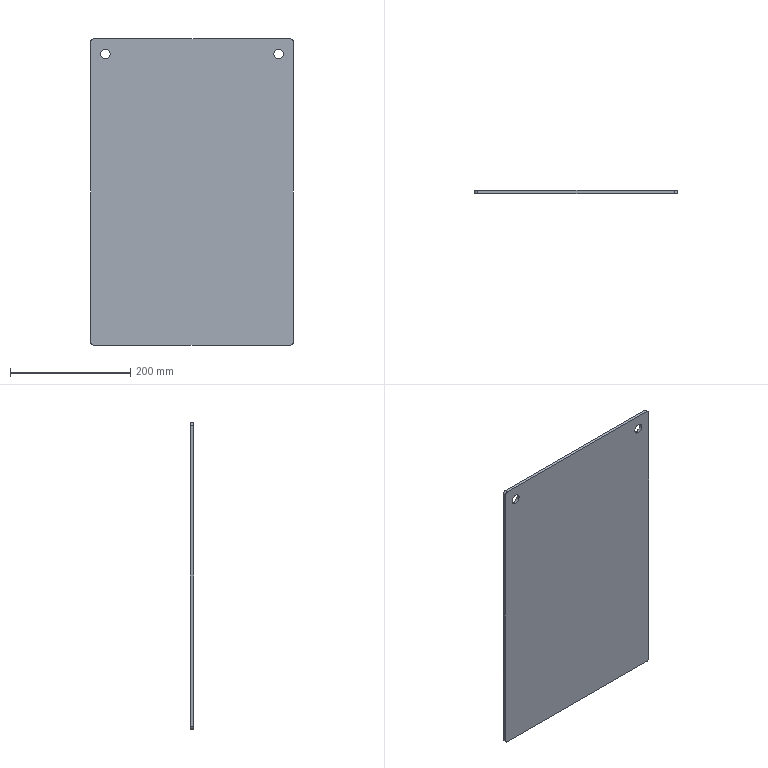Component | SolidWorks | 008FrameTopCoverPlate-1 | 1 solid | 14 faces | box 338 x 5 x 510 mm | volume 859661 mm3 | plane 6 | cone 4 | cylinder 4 | commonest cylinder face diameters 10 x4 | material Plain Carbon Steel
build123d program:
from build123d import *

# Parameters (mm, degrees)
SKETCH1_W                        = 510
SKETCH1_H                        = 338
BOSS_EXTRUDE1_DEPTH              = 5
FILLET1_R                        = 5
F_1_2_RC_TAPPED_HOLE1_AT_2_COUNT = 2
F_1_2_RC_TAPPED_HOLE1_AT_2_PITCH = 289


with BuildPart() as part:
    # Sketch1 → Boss-Extrude1 (new body)
    with BuildSketch(Plane.XY):
        Rectangle(SKETCH1_W, SKETCH1_H)
    extrude(amount=BOSS_EXTRUDE1_DEPTH)

    # Fillet1
    fillet1_edges = [part.edges().sort_by_distance(p)[0] for p in [
        (255, -169, 2.5),
        (-255, -169, 2.5),
        (-255, 169, 2.5),
        (255, 169, 2.5),
    ]]
    fillet(fillet1_edges, radius=FILLET1_R)

    # Sketch2 → 1_2 Rc Tapped Hole1 (revolve, cut)
    with BuildSketch(Plane(origin=(-230, -144.5, 0), x_dir=(0, 1, 0), z_dir=(1, 0, 0))):
        Polygon((0, 0), (0, 29.328), (8.75, 24.07), (8.75, 15), (7.847, 15), (8.316, 0), align=None)
    f_1_2_rc_tapped_hole1 = revolve(axis=Axis((-230, -144.5, -6.35), (0, 0, 1)), mode=Mode.SUBTRACT)

    # 1_2 Rc Tapped Hole1 at 2: 1_2 Rc Tapped Hole1 ×2
    with Locations(*[(0, i * F_1_2_RC_TAPPED_HOLE1_AT_2_PITCH, 0) for i in range(1, F_1_2_RC_TAPPED_HOLE1_AT_2_COUNT)]):
        add(f_1_2_rc_tapped_hole1, mode=Mode.SUBTRACT)


solid = part.part

# Placed as in the assembly
solid = solid.moved(Location((130, 1377, -260), (90, 0, -90)))
STEP:
#1=COLOUR_RGB('',0.7922,0.8196,0.9333);
#2=FILL_AREA_STYLE_COLOUR('',#1);
#3=FILL_AREA_STYLE('',(#2));
#4=SURFACE_STYLE_FILL_AREA(#3);
#5=SURFACE_SIDE_STYLE('',(#4));
#6=SURFACE_STYLE_USAGE(.BOTH.,#5);
#7=PRESENTATION_STYLE_ASSIGNMENT((#6));
#8=CARTESIAN_POINT('',(-0.5709,54.016,-1.502));
#9=VERTEX_POINT('',#8);
#10=CARTESIAN_POINT('',(-0.5709,54.016,-0.8599));
#11=VERTEX_POINT('',#10);
#12=CARTESIAN_POINT('',(-0.5709,54.016,-1.181));
#13=DIRECTION('',(0.,1.,0.));
#14=DIRECTION('',(-0.,0.,1.));
#15=AXIS2_PLACEMENT_3D('',#12,#13,#14);
#16=CIRCLE('',#15,0.3212);
#17=EDGE_CURVE('',#9,#11,#16,.T.);
#18=ORIENTED_EDGE('',*,*,#17,.F.);
#19=CARTESIAN_POINT('',(-0.5709,54.213,-1.508));
#20=VERTEX_POINT('',#19);
#21=CARTESIAN_POINT('',(-0.5709,54.213,-1.508));
#22=DIRECTION('',(0.,0.9995,-0.0312));
#23=VECTOR('',#22,39.37);
#24=LINE('',#21,#23);
#25=EDGE_CURVE('',#9,#20,#24,.T.);
#26=ORIENTED_EDGE('',*,*,#25,.T.);
#27=CARTESIAN_POINT('',(-0.5709,54.213,-0.8537));
#28=VERTEX_POINT('',#27);
#29=CARTESIAN_POINT('',(-0.5709,54.213,-1.181));
#30=DIRECTION('',(0.,1.,0.));
#31=DIRECTION('',(-0.,0.,1.));
#32=AXIS2_PLACEMENT_3D('',#29,#30,#31);
#33=CIRCLE('',#32,0.3274);
#34=EDGE_CURVE('',#20,#28,#33,.T.);
#35=ORIENTED_EDGE('',*,*,#34,.T.);
#36=CARTESIAN_POINT('',(-0.5709,54.213,-0.8537));
#37=DIRECTION('',(-0.,0.9995,0.0312));
#38=VECTOR('',#37,39.37);
#39=LINE('',#36,#38);
#40=EDGE_CURVE('',#11,#28,#39,.T.);
#41=ORIENTED_EDGE('',*,*,#40,.F.);
#42=EDGE_LOOP('',(#18,#26,#35,#41));
#43=FACE_OUTER_BOUND('',#42,.T.);
#44=CARTESIAN_POINT('',(-0.5709,54.213,-1.181));
#45=DIRECTION('',(0.,1.,0.));
#46=DIRECTION('',(-0.,0.,1.));
#47=AXIS2_PLACEMENT_3D('',#44,#45,#46);
#48=CONICAL_SURFACE('',#47,0.3274,0.03121);
#49=ADVANCED_FACE('',(#43),#48,.F.);
#50=CARTESIAN_POINT('',(10.807,54.016,-1.502));
#51=VERTEX_POINT('',#50);
#52=CARTESIAN_POINT('',(10.807,54.016,-0.8599));
#53=VERTEX_POINT('',#52);
#54=CARTESIAN_POINT('',(10.807,54.016,-1.181));
#55=DIRECTION('',(0.,1.,0.));
#56=DIRECTION('',(0.,0.,1.));
#57=AXIS2_PLACEMENT_3D('',#54,#55,#56);
#58=CIRCLE('',#57,0.3212);
#59=EDGE_CURVE('',#51,#53,#58,.T.);
#60=ORIENTED_EDGE('',*,*,#59,.F.);
#61=CARTESIAN_POINT('',(10.807,54.213,-1.508));
#62=VERTEX_POINT('',#61);
#63=CARTESIAN_POINT('',(10.807,54.213,-1.508));
#64=DIRECTION('',(0.,0.9995,-0.0312));
#65=VECTOR('',#64,39.37);
#66=LINE('',#63,#65);
#67=EDGE_CURVE('',#51,#62,#66,.T.);
#68=ORIENTED_EDGE('',*,*,#67,.T.);
#69=CARTESIAN_POINT('',(10.807,54.213,-0.8537));
#70=VERTEX_POINT('',#69);
#71=CARTESIAN_POINT('',(10.807,54.213,-1.181));
#72=DIRECTION('',(0.,1.,0.));
#73=DIRECTION('',(0.,0.,1.));
#74=AXIS2_PLACEMENT_3D('',#71,#72,#73);
#75=CIRCLE('',#74,0.3274);
#76=EDGE_CURVE('',#62,#70,#75,.T.);
#77=ORIENTED_EDGE('',*,*,#76,.T.);
#78=CARTESIAN_POINT('',(10.807,54.213,-0.8537));
#79=DIRECTION('',(-0.,0.9995,0.0312));
#80=VECTOR('',#79,39.37);
#81=LINE('',#78,#80);
#82=EDGE_CURVE('',#53,#70,#81,.T.);
#83=ORIENTED_EDGE('',*,*,#82,.F.);
#84=EDGE_LOOP('',(#60,#68,#77,#83));
#85=FACE_OUTER_BOUND('',#84,.T.);
#86=CARTESIAN_POINT('',(10.807,54.213,-1.181));
#87=DIRECTION('',(0.,1.,0.));
#88=DIRECTION('',(0.,0.,1.));
#89=AXIS2_PLACEMENT_3D('',#86,#87,#88);
#90=CONICAL_SURFACE('',#89,0.3274,0.03121);
#91=ADVANCED_FACE('',(#85),#90,.F.);
#92=CARTESIAN_POINT('',(-1.339,54.016,-20.276));
#93=VERTEX_POINT('',#92);
#94=CARTESIAN_POINT('',(11.575,54.016,-20.276));
#95=VERTEX_POINT('',#94);
#96=CARTESIAN_POINT('',(-1.535,54.016,-20.276));
#97=DIRECTION('',(1.,0.,0.));
#98=VECTOR('',#97,39.37);
#99=LINE('',#96,#98);
#100=EDGE_CURVE('',#93,#95,#99,.T.);
#101=ORIENTED_EDGE('',*,*,#100,.F.);
#102=CARTESIAN_POINT('',(-1.339,54.213,-20.276));
#103=VERTEX_POINT('',#102);
#104=CARTESIAN_POINT('',(-1.339,54.016,-20.276));
#105=DIRECTION('',(0.,1.,0.));
#106=VECTOR('',#105,39.37);
#107=LINE('',#104,#106);
#108=EDGE_CURVE('',#93,#103,#107,.T.);
#109=ORIENTED_EDGE('',*,*,#108,.T.);
#110=CARTESIAN_POINT('',(11.575,54.213,-20.276));
#111=VERTEX_POINT('',#110);
#112=CARTESIAN_POINT('',(-1.535,54.213,-20.276));
#113=DIRECTION('',(1.,0.,0.));
#114=VECTOR('',#113,39.37);
#115=LINE('',#112,#114);
#116=EDGE_CURVE('',#103,#111,#115,.T.);
#117=ORIENTED_EDGE('',*,*,#116,.T.);
#118=CARTESIAN_POINT('',(11.575,54.016,-20.276));
#119=DIRECTION('',(0.,-1.,0.));
#120=VECTOR('',#119,39.37);
#121=LINE('',#118,#120);
#122=EDGE_CURVE('',#111,#95,#121,.T.);
#123=ORIENTED_EDGE('',*,*,#122,.T.);
#124=EDGE_LOOP('',(#101,#109,#117,#123));
#125=FACE_OUTER_BOUND('',#124,.T.);
#126=CARTESIAN_POINT('',(-1.535,54.016,-20.276));
#127=DIRECTION('',(-0.,0.,1.));
#128=DIRECTION('',(0.,-1.,0.));
#129=AXIS2_PLACEMENT_3D('',#126,#127,#128);
#130=PLANE('',#129);
#131=ADVANCED_FACE('',(#125),#130,.F.);
#132=CARTESIAN_POINT('',(11.772,54.213,-20.079));
#133=VERTEX_POINT('',#132);
#134=CARTESIAN_POINT('',(11.772,54.213,-0.3937));
#135=VERTEX_POINT('',#134);
#136=CARTESIAN_POINT('',(11.772,54.213,-0.1969));
#137=DIRECTION('',(-0.,0.,1.));
#138=VECTOR('',#137,39.37);
#139=LINE('',#136,#138);
#140=EDGE_CURVE('',#133,#135,#139,.T.);
#141=ORIENTED_EDGE('',*,*,#140,.T.);
#142=CARTESIAN_POINT('',(11.772,54.016,-0.3937));
#143=VERTEX_POINT('',#142);
#144=CARTESIAN_POINT('',(11.772,54.016,-0.3937));
#145=DIRECTION('',(0.,-1.,0.));
#146=VECTOR('',#145,39.37);
#147=LINE('',#144,#146);
#148=EDGE_CURVE('',#135,#143,#147,.T.);
#149=ORIENTED_EDGE('',*,*,#148,.T.);
#150=CARTESIAN_POINT('',(11.772,54.016,-20.079));
#151=VERTEX_POINT('',#150);
#152=CARTESIAN_POINT('',(11.772,54.016,-0.1969));
#153=DIRECTION('',(-0.,0.,1.));
#154=VECTOR('',#153,39.37);
#155=LINE('',#152,#154);
#156=EDGE_CURVE('',#151,#143,#155,.T.);
#157=ORIENTED_EDGE('',*,*,#156,.F.);
#158=CARTESIAN_POINT('',(11.772,54.016,-20.079));
#159=DIRECTION('',(0.,1.,0.));
#160=VECTOR('',#159,39.37);
#161=LINE('',#158,#160);
#162=EDGE_CURVE('',#151,#133,#161,.T.);
#163=ORIENTED_EDGE('',*,*,#162,.T.);
#164=EDGE_LOOP('',(#141,#149,#157,#163));
#165=FACE_OUTER_BOUND('',#164,.T.);
#166=CARTESIAN_POINT('',(11.772,54.016,-0.1969));
#167=DIRECTION('',(-1.,0.,-0.));
#168=DIRECTION('',(0.,1.,0.));
#169=AXIS2_PLACEMENT_3D('',#166,#167,#168);
#170=PLANE('',#169);
#171=ADVANCED_FACE('',(#165),#170,.F.);
#172=CARTESIAN_POINT('',(11.575,54.213,-0.1969));
#173=VERTEX_POINT('',#172);
#174=CARTESIAN_POINT('',(-1.339,54.213,-0.1969));
#175=VERTEX_POINT('',#174);
#176=CARTESIAN_POINT('',(-1.535,54.213,-0.1969));
#177=DIRECTION('',(-1.,0.,-0.));
#178=VECTOR('',#177,39.37);
#179=LINE('',#176,#178);
#180=EDGE_CURVE('',#173,#175,#179,.T.);
#181=ORIENTED_EDGE('',*,*,#180,.T.);
#182=CARTESIAN_POINT('',(-1.339,54.016,-0.1969));
#183=VERTEX_POINT('',#182);
#184=CARTESIAN_POINT('',(-1.339,54.016,-0.1969));
#185=DIRECTION('',(0.,-1.,0.));
#186=VECTOR('',#185,39.37);
#187=LINE('',#184,#186);
#188=EDGE_CURVE('',#175,#183,#187,.T.);
#189=ORIENTED_EDGE('',*,*,#188,.T.);
#190=CARTESIAN_POINT('',(11.575,54.016,-0.1969));
#191=VERTEX_POINT('',#190);
#192=CARTESIAN_POINT('',(-1.535,54.016,-0.1969));
#193=DIRECTION('',(-1.,0.,-0.));
#194=VECTOR('',#193,39.37);
#195=LINE('',#192,#194);
#196=EDGE_CURVE('',#191,#183,#195,.T.);
#197=ORIENTED_EDGE('',*,*,#196,.F.);
#198=CARTESIAN_POINT('',(11.575,54.016,-0.1969));
#199=DIRECTION('',(0.,1.,0.));
#200=VECTOR('',#199,39.37);
#201=LINE('',#198,#200);
#202=EDGE_CURVE('',#191,#173,#201,.T.);
#203=ORIENTED_EDGE('',*,*,#202,.T.);
#204=EDGE_LOOP('',(#181,#189,#197,#203));
#205=FACE_OUTER_BOUND('',#204,.T.);
#206=CARTESIAN_POINT('',(-1.535,54.016,-0.1969));
#207=DIRECTION('',(0.,0.,-1.));
#208=DIRECTION('',(0.,1.,0.));
#209=AXIS2_PLACEMENT_3D('',#206,#207,#208);
#210=PLANE('',#209);
#211=ADVANCED_FACE('',(#205),#210,.F.);
#212=CARTESIAN_POINT('',(-1.535,54.213,-0.3937));
#213=VERTEX_POINT('',#212);
#214=CARTESIAN_POINT('',(-1.535,54.213,-20.079));
#215=VERTEX_POINT('',#214);
#216=CARTESIAN_POINT('',(-1.535,54.213,-0.1969));
#217=DIRECTION('',(0.,0.,-1.));
#218=VECTOR('',#217,39.37);
#219=LINE('',#216,#218);
#220=EDGE_CURVE('',#213,#215,#219,.T.);
#221=ORIENTED_EDGE('',*,*,#220,.T.);
#222=CARTESIAN_POINT('',(-1.535,54.016,-20.079));
#223=VERTEX_POINT('',#222);
#224=CARTESIAN_POINT('',(-1.535,54.016,-20.079));
#225=DIRECTION('',(0.,-1.,0.));
#226=VECTOR('',#225,39.37);
#227=LINE('',#224,#226);
#228=EDGE_CURVE('',#215,#223,#227,.T.);
#229=ORIENTED_EDGE('',*,*,#228,.T.);
#230=CARTESIAN_POINT('',(-1.535,54.016,-0.3937));
#231=VERTEX_POINT('',#230);
#232=CARTESIAN_POINT('',(-1.535,54.016,-0.1969));
#233=DIRECTION('',(0.,0.,-1.));
#234=VECTOR('',#233,39.37);
#235=LINE('',#232,#234);
#236=EDGE_CURVE('',#231,#223,#235,.T.);
#237=ORIENTED_EDGE('',*,*,#236,.F.);
#238=CARTESIAN_POINT('',(-1.535,54.016,-0.3937));
#239=DIRECTION('',(0.,1.,0.));
#240=VECTOR('',#239,39.37);
#241=LINE('',#238,#240);
#242=EDGE_CURVE('',#231,#213,#241,.T.);
#243=ORIENTED_EDGE('',*,*,#242,.T.);
#244=EDGE_LOOP('',(#221,#229,#237,#243));
#245=FACE_OUTER_BOUND('',#244,.T.);
#246=CARTESIAN_POINT('',(-1.535,54.016,-0.1969));
#247=DIRECTION('',(1.,0.,0.));
#248=DIRECTION('',(0.,-1.,0.));
#249=AXIS2_PLACEMENT_3D('',#246,#247,#248);
#250=PLANE('',#249);
#251=ADVANCED_FACE('',(#245),#250,.F.);
#252=CARTESIAN_POINT('',(-0.5709,54.016,-1.181));
#253=DIRECTION('',(0.,1.,0.));
#254=DIRECTION('',(-0.,0.,1.));
#255=AXIS2_PLACEMENT_3D('',#252,#253,#254);
#256=CIRCLE('',#255,0.3212);
#257=EDGE_CURVE('',#11,#9,#256,.T.);
#258=ORIENTED_EDGE('',*,*,#257,.T.);
#259=ORIENTED_EDGE('',*,*,#17,.T.);
#260=EDGE_LOOP('',(#258,#259));
#261=FACE_BOUND('',#260,.T.);
#262=CARTESIAN_POINT('',(10.807,54.016,-1.181));
#263=DIRECTION('',(0.,1.,0.));
#264=DIRECTION('',(0.,0.,1.));
#265=AXIS2_PLACEMENT_3D('',#262,#263,#264);
#266=CIRCLE('',#265,0.3212);
#267=EDGE_CURVE('',#53,#51,#266,.T.);
#268=ORIENTED_EDGE('',*,*,#267,.T.);
#269=ORIENTED_EDGE('',*,*,#59,.T.);
#270=EDGE_LOOP('',(#268,#269));
#271=FACE_BOUND('',#270,.T.);
#272=ORIENTED_EDGE('',*,*,#236,.T.);
#273=CARTESIAN_POINT('',(-1.339,54.016,-20.079));
#274=DIRECTION('',(0.,-1.,0.));
#275=DIRECTION('',(0.,0.,1.));
#276=AXIS2_PLACEMENT_3D('',#273,#274,#275);
#277=CIRCLE('',#276,0.1969);
#278=EDGE_CURVE('',#223,#93,#277,.T.);
#279=ORIENTED_EDGE('',*,*,#278,.T.);
#280=ORIENTED_EDGE('',*,*,#100,.T.);
#281=CARTESIAN_POINT('',(11.575,54.016,-20.079));
#282=DIRECTION('',(0.,-1.,0.));
#283=DIRECTION('',(0.,0.,1.));
#284=AXIS2_PLACEMENT_3D('',#281,#282,#283);
#285=CIRCLE('',#284,0.1969);
#286=EDGE_CURVE('',#95,#151,#285,.T.);
#287=ORIENTED_EDGE('',*,*,#286,.T.);
#288=ORIENTED_EDGE('',*,*,#156,.T.);
#289=CARTESIAN_POINT('',(11.575,54.016,-0.3937));
#290=DIRECTION('',(0.,-1.,0.));
#291=DIRECTION('',(0.,0.,1.));
#292=AXIS2_PLACEMENT_3D('',#289,#290,#291);
#293=CIRCLE('',#292,0.1969);
#294=EDGE_CURVE('',#143,#191,#293,.T.);
#295=ORIENTED_EDGE('',*,*,#294,.T.);
#296=ORIENTED_EDGE('',*,*,#196,.T.);
#297=CARTESIAN_POINT('',(-1.339,54.016,-0.3937));
#298=DIRECTION('',(0.,-1.,0.));
#299=DIRECTION('',(0.,0.,1.));
#300=AXIS2_PLACEMENT_3D('',#297,#298,#299);
#301=CIRCLE('',#300,0.1969);
#302=EDGE_CURVE('',#183,#231,#301,.T.);
#303=ORIENTED_EDGE('',*,*,#302,.T.);
#304=EDGE_LOOP('',(#272,#279,#280,#287,#288,#295,#296,#303));
#305=FACE_OUTER_BOUND('',#304,.T.);
#306=CARTESIAN_POINT('',(11.772,54.016,-20.276));
#307=DIRECTION('',(0.,1.,0.));
#308=DIRECTION('',(-0.,0.,1.));
#309=AXIS2_PLACEMENT_3D('',#306,#307,#308);
#310=PLANE('',#309);
#311=ADVANCED_FACE('',(#261,#271,#305),#310,.F.);
#312=CARTESIAN_POINT('',(-0.5709,54.213,-1.181));
#313=DIRECTION('',(0.,1.,0.));
#314=DIRECTION('',(-0.,0.,1.));
#315=AXIS2_PLACEMENT_3D('',#312,#313,#314);
#316=CIRCLE('',#315,0.3274);
#317=EDGE_CURVE('',#28,#20,#316,.T.);
#318=ORIENTED_EDGE('',*,*,#317,.F.);
#319=ORIENTED_EDGE('',*,*,#34,.F.);
#320=EDGE_LOOP('',(#318,#319));
#321=FACE_BOUND('',#320,.T.);
#322=CARTESIAN_POINT('',(10.807,54.213,-1.181));
#323=DIRECTION('',(0.,1.,0.));
#324=DIRECTION('',(0.,0.,1.));
#325=AXIS2_PLACEMENT_3D('',#322,#323,#324);
#326=CIRCLE('',#325,0.3274);
#327=EDGE_CURVE('',#70,#62,#326,.T.);
#328=ORIENTED_EDGE('',*,*,#327,.F.);
#329=ORIENTED_EDGE('',*,*,#76,.F.);
#330=EDGE_LOOP('',(#328,#329));
#331=FACE_BOUND('',#330,.T.);
#332=ORIENTED_EDGE('',*,*,#116,.F.);
#333=CARTESIAN_POINT('',(-1.339,54.213,-20.079));
#334=DIRECTION('',(0.,1.,0.));
#335=DIRECTION('',(0.,0.,1.));
#336=AXIS2_PLACEMENT_3D('',#333,#334,#335);
#337=CIRCLE('',#336,0.1969);
#338=EDGE_CURVE('',#103,#215,#337,.T.);
#339=ORIENTED_EDGE('',*,*,#338,.T.);
#340=ORIENTED_EDGE('',*,*,#220,.F.);
#341=CARTESIAN_POINT('',(-1.339,54.213,-0.3937));
#342=DIRECTION('',(0.,1.,0.));
#343=DIRECTION('',(0.,0.,1.));
#344=AXIS2_PLACEMENT_3D('',#341,#342,#343);
#345=CIRCLE('',#344,0.1969);
#346=EDGE_CURVE('',#213,#175,#345,.T.);
#347=ORIENTED_EDGE('',*,*,#346,.T.);
#348=ORIENTED_EDGE('',*,*,#180,.F.);
#349=CARTESIAN_POINT('',(11.575,54.213,-0.3937));
#350=DIRECTION('',(0.,1.,0.));
#351=DIRECTION('',(0.,0.,1.));
#352=AXIS2_PLACEMENT_3D('',#349,#350,#351);
#353=CIRCLE('',#352,0.1969);
#354=EDGE_CURVE('',#173,#135,#353,.T.);
#355=ORIENTED_EDGE('',*,*,#354,.T.);
#356=ORIENTED_EDGE('',*,*,#140,.F.);
#357=CARTESIAN_POINT('',(11.575,54.213,-20.079));
#358=DIRECTION('',(0.,1.,0.));
#359=DIRECTION('',(0.,0.,1.));
#360=AXIS2_PLACEMENT_3D('',#357,#358,#359);
#361=CIRCLE('',#360,0.1969);
#362=EDGE_CURVE('',#133,#111,#361,.T.);
#363=ORIENTED_EDGE('',*,*,#362,.T.);
#364=EDGE_LOOP('',(#332,#339,#340,#347,#348,#355,#356,#363));
#365=FACE_OUTER_BOUND('',#364,.T.);
#366=CARTESIAN_POINT('',(11.772,54.213,-20.276));
#367=DIRECTION('',(0.,1.,0.));
#368=DIRECTION('',(-0.,0.,1.));
#369=AXIS2_PLACEMENT_3D('',#366,#367,#368);
#370=PLANE('',#369);
#371=ADVANCED_FACE('',(#321,#331,#365),#370,.T.);
#372=ORIENTED_EDGE('',*,*,#278,.F.);
#373=ORIENTED_EDGE('',*,*,#228,.F.);
#374=ORIENTED_EDGE('',*,*,#338,.F.);
#375=ORIENTED_EDGE('',*,*,#108,.F.);
#376=EDGE_LOOP('',(#372,#373,#374,#375));
#377=FACE_OUTER_BOUND('',#376,.T.);
#378=CARTESIAN_POINT('',(-1.339,54.016,-20.079));
#379=DIRECTION('',(0.,1.,0.));
#380=DIRECTION('',(0.,0.,1.));
#381=AXIS2_PLACEMENT_3D('',#378,#379,#380);
#382=CYLINDRICAL_SURFACE('',#381,0.1969);
#383=ADVANCED_FACE('',(#377),#382,.T.);
#384=ORIENTED_EDGE('',*,*,#302,.F.);
#385=ORIENTED_EDGE('',*,*,#188,.F.);
#386=ORIENTED_EDGE('',*,*,#346,.F.);
#387=ORIENTED_EDGE('',*,*,#242,.F.);
#388=EDGE_LOOP('',(#384,#385,#386,#387));
#389=FACE_OUTER_BOUND('',#388,.T.);
#390=CARTESIAN_POINT('',(-1.339,54.016,-0.3937));
#391=DIRECTION('',(0.,1.,0.));
#392=DIRECTION('',(0.,0.,1.));
#393=AXIS2_PLACEMENT_3D('',#390,#391,#392);
#394=CYLINDRICAL_SURFACE('',#393,0.1969);
#395=ADVANCED_FACE('',(#389),#394,.T.);
#396=ORIENTED_EDGE('',*,*,#294,.F.);
#397=ORIENTED_EDGE('',*,*,#148,.F.);
#398=ORIENTED_EDGE('',*,*,#354,.F.);
#399=ORIENTED_EDGE('',*,*,#202,.F.);
#400=EDGE_LOOP('',(#396,#397,#398,#399));
#401=FACE_OUTER_BOUND('',#400,.T.);
#402=CARTESIAN_POINT('',(11.575,54.016,-0.3937));
#403=DIRECTION('',(0.,1.,0.));
#404=DIRECTION('',(0.,0.,1.));
#405=AXIS2_PLACEMENT_3D('',#402,#403,#404);
#406=CYLINDRICAL_SURFACE('',#405,0.1969);
#407=ADVANCED_FACE('',(#401),#406,.T.);
#408=ORIENTED_EDGE('',*,*,#286,.F.);
#409=ORIENTED_EDGE('',*,*,#122,.F.);
#410=ORIENTED_EDGE('',*,*,#362,.F.);
#411=ORIENTED_EDGE('',*,*,#162,.F.);
#412=EDGE_LOOP('',(#408,#409,#410,#411));
#413=FACE_OUTER_BOUND('',#412,.T.);
#414=CARTESIAN_POINT('',(11.575,54.016,-20.079));
#415=DIRECTION('',(0.,1.,0.));
#416=DIRECTION('',(0.,0.,1.));
#417=AXIS2_PLACEMENT_3D('',#414,#415,#416);
#418=CYLINDRICAL_SURFACE('',#417,0.1969);
#419=ADVANCED_FACE('',(#413),#418,.T.);
#420=ORIENTED_EDGE('',*,*,#67,.F.);
#421=ORIENTED_EDGE('',*,*,#267,.F.);
#422=ORIENTED_EDGE('',*,*,#82,.T.);
#423=ORIENTED_EDGE('',*,*,#327,.T.);
#424=EDGE_LOOP('',(#420,#421,#422,#423));
#425=FACE_OUTER_BOUND('',#424,.T.);
#426=CARTESIAN_POINT('',(10.807,54.213,-1.181));
#427=DIRECTION('',(0.,1.,0.));
#428=DIRECTION('',(0.,0.,1.));
#429=AXIS2_PLACEMENT_3D('',#426,#427,#428);
#430=CONICAL_SURFACE('',#429,0.3274,0.03121);
#431=ADVANCED_FACE('',(#425),#430,.F.);
#432=ORIENTED_EDGE('',*,*,#25,.F.);
#433=ORIENTED_EDGE('',*,*,#257,.F.);
#434=ORIENTED_EDGE('',*,*,#40,.T.);
#435=ORIENTED_EDGE('',*,*,#317,.T.);
#436=EDGE_LOOP('',(#432,#433,#434,#435));
#437=FACE_OUTER_BOUND('',#436,.T.);
#438=CARTESIAN_POINT('',(-0.5709,54.213,-1.181));
#439=DIRECTION('',(0.,1.,0.));
#440=DIRECTION('',(-0.,0.,1.));
#441=AXIS2_PLACEMENT_3D('',#438,#439,#440);
#442=CONICAL_SURFACE('',#441,0.3274,0.03121);
#443=ADVANCED_FACE('',(#437),#442,.F.);
#444=CLOSED_SHELL('',(#49,#91,#131,#171,#211,#251,#311,#371,#383,#395,#407,#419,#431,#443));
#445=MANIFOLD_SOLID_BREP('',#444);
#446=STYLED_ITEM('',(#7),#445);
#447=PRESENTATION_LAYER_ASSIGNMENT('','',(#446));
#448=(LENGTH_UNIT()NAMED_UNIT(*)SI_UNIT($,.METRE.));
#449=LENGTH_MEASURE_WITH_UNIT(LENGTH_MEASURE(0.0254),#448);
#450=DIMENSIONAL_EXPONENTS(1.,0.,0.,0.,0.,0.,0.);
#451=(CONVERSION_BASED_UNIT('',#449)LENGTH_UNIT()NAMED_UNIT(#450));
#452=UNCERTAINTY_MEASURE_WITH_UNIT(LENGTH_MEASURE(0.00001),#451,'','');
#453=(NAMED_UNIT(*)PLANE_ANGLE_UNIT()SI_UNIT($,.RADIAN.));
#454=(NAMED_UNIT(*)SI_UNIT($,.STERADIAN.)SOLID_ANGLE_UNIT());
#455=(GEOMETRIC_REPRESENTATION_CONTEXT(3)GLOBAL_UNCERTAINTY_ASSIGNED_CONTEXT((#452))GLOBAL_UNIT_ASSIGNED_CONTEXT((#451,#453,#454))REPRESENTATION_CONTEXT('',''));
#456=MECHANICAL_DESIGN_GEOMETRIC_PRESENTATION_REPRESENTATION('',(#446),#455);
#457=CARTESIAN_POINT('',(0.,0.,0.));
#458=DIRECTION('',(0.,0.,1.));
#459=DIRECTION('',(1.,0.,0.));
#460=AXIS2_PLACEMENT_3D('',#457,#458,#459);
#461=(LENGTH_UNIT()NAMED_UNIT(*)SI_UNIT($,.METRE.));
#462=LENGTH_MEASURE_WITH_UNIT(LENGTH_MEASURE(0.0254),#461);
#463=DIMENSIONAL_EXPONENTS(1.,0.,0.,0.,0.,0.,0.);
#464=(CONVERSION_BASED_UNIT('',#462)LENGTH_UNIT()NAMED_UNIT(#463));
#465=UNCERTAINTY_MEASURE_WITH_UNIT(LENGTH_MEASURE(0.00001),#464,'','');
#466=(NAMED_UNIT(*)PLANE_ANGLE_UNIT()SI_UNIT($,.RADIAN.));
#467=(NAMED_UNIT(*)SI_UNIT($,.STERADIAN.)SOLID_ANGLE_UNIT());
#468=(GEOMETRIC_REPRESENTATION_CONTEXT(3)GLOBAL_UNCERTAINTY_ASSIGNED_CONTEXT((#465))GLOBAL_UNIT_ASSIGNED_CONTEXT((#464,#466,#467))REPRESENTATION_CONTEXT('',''));
#469=ADVANCED_BREP_SHAPE_REPRESENTATION('',(#445,#460),#468);